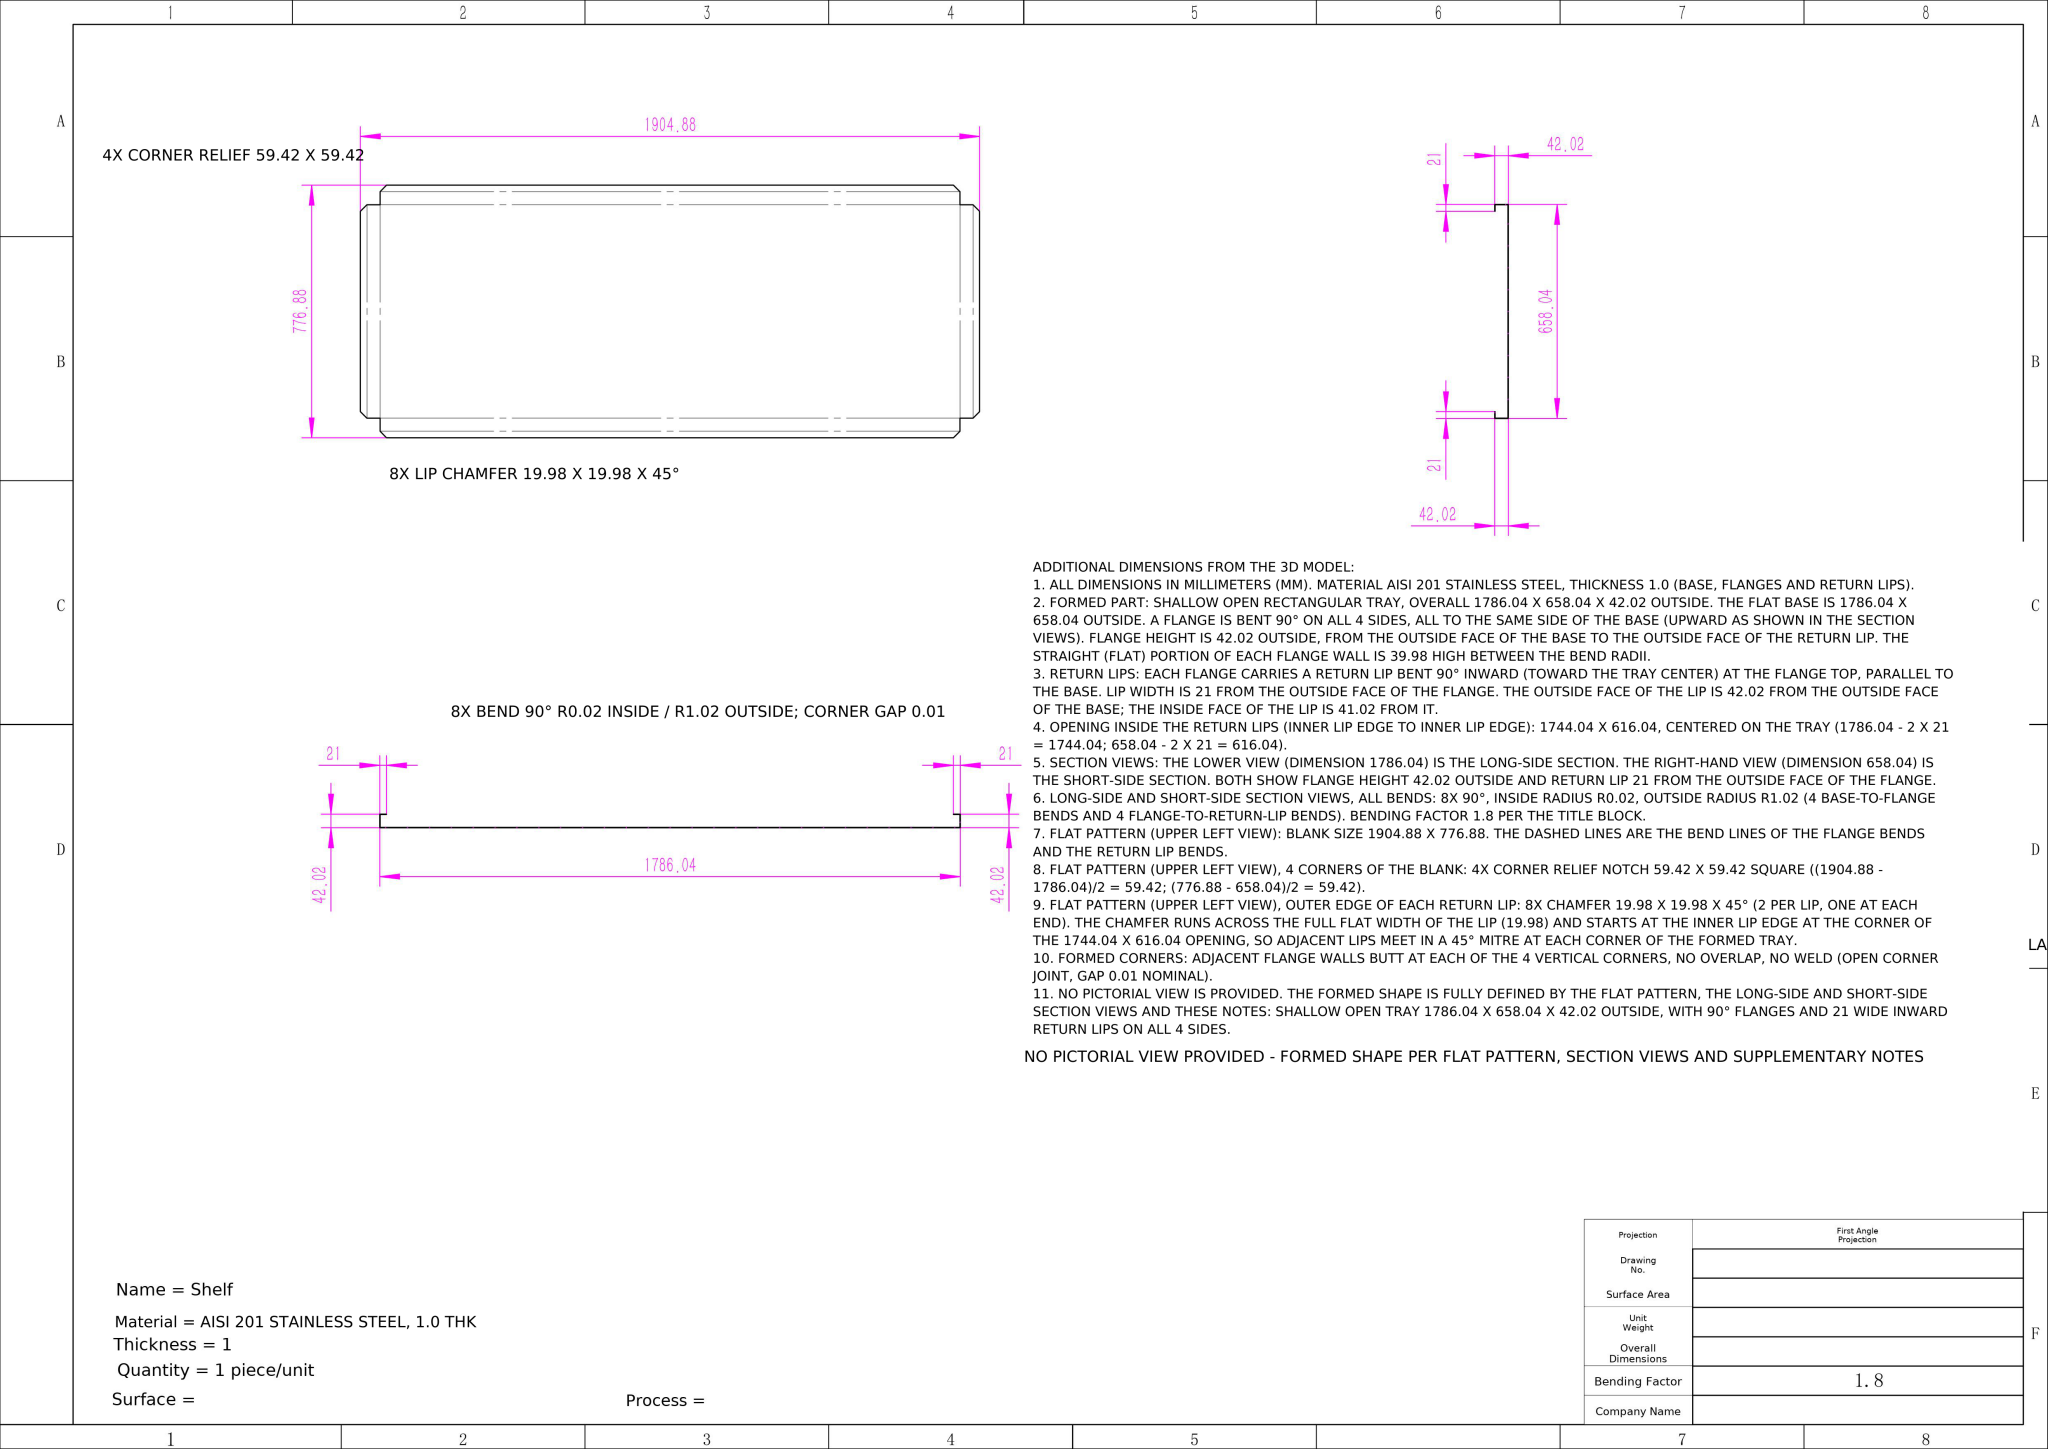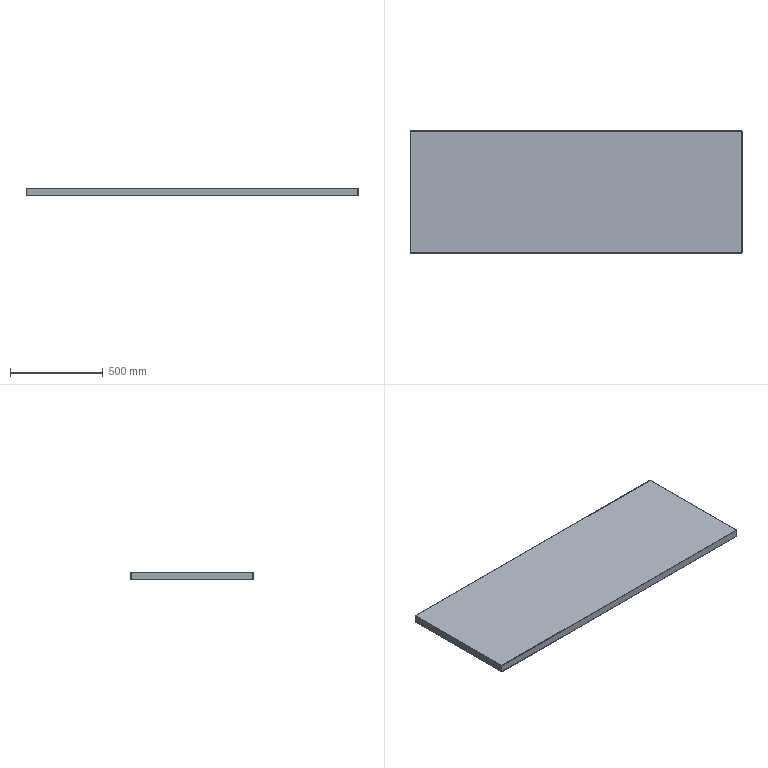Part | NX | mm | 1 solid | 70 faces | box 1786.04 x 658.04 x 42.02 mm | volume 1469287 mm3 | plane 38 | spline 16 | cylinder 16 | commonest cylinder face diameters 2.04 x8 0.04 x8